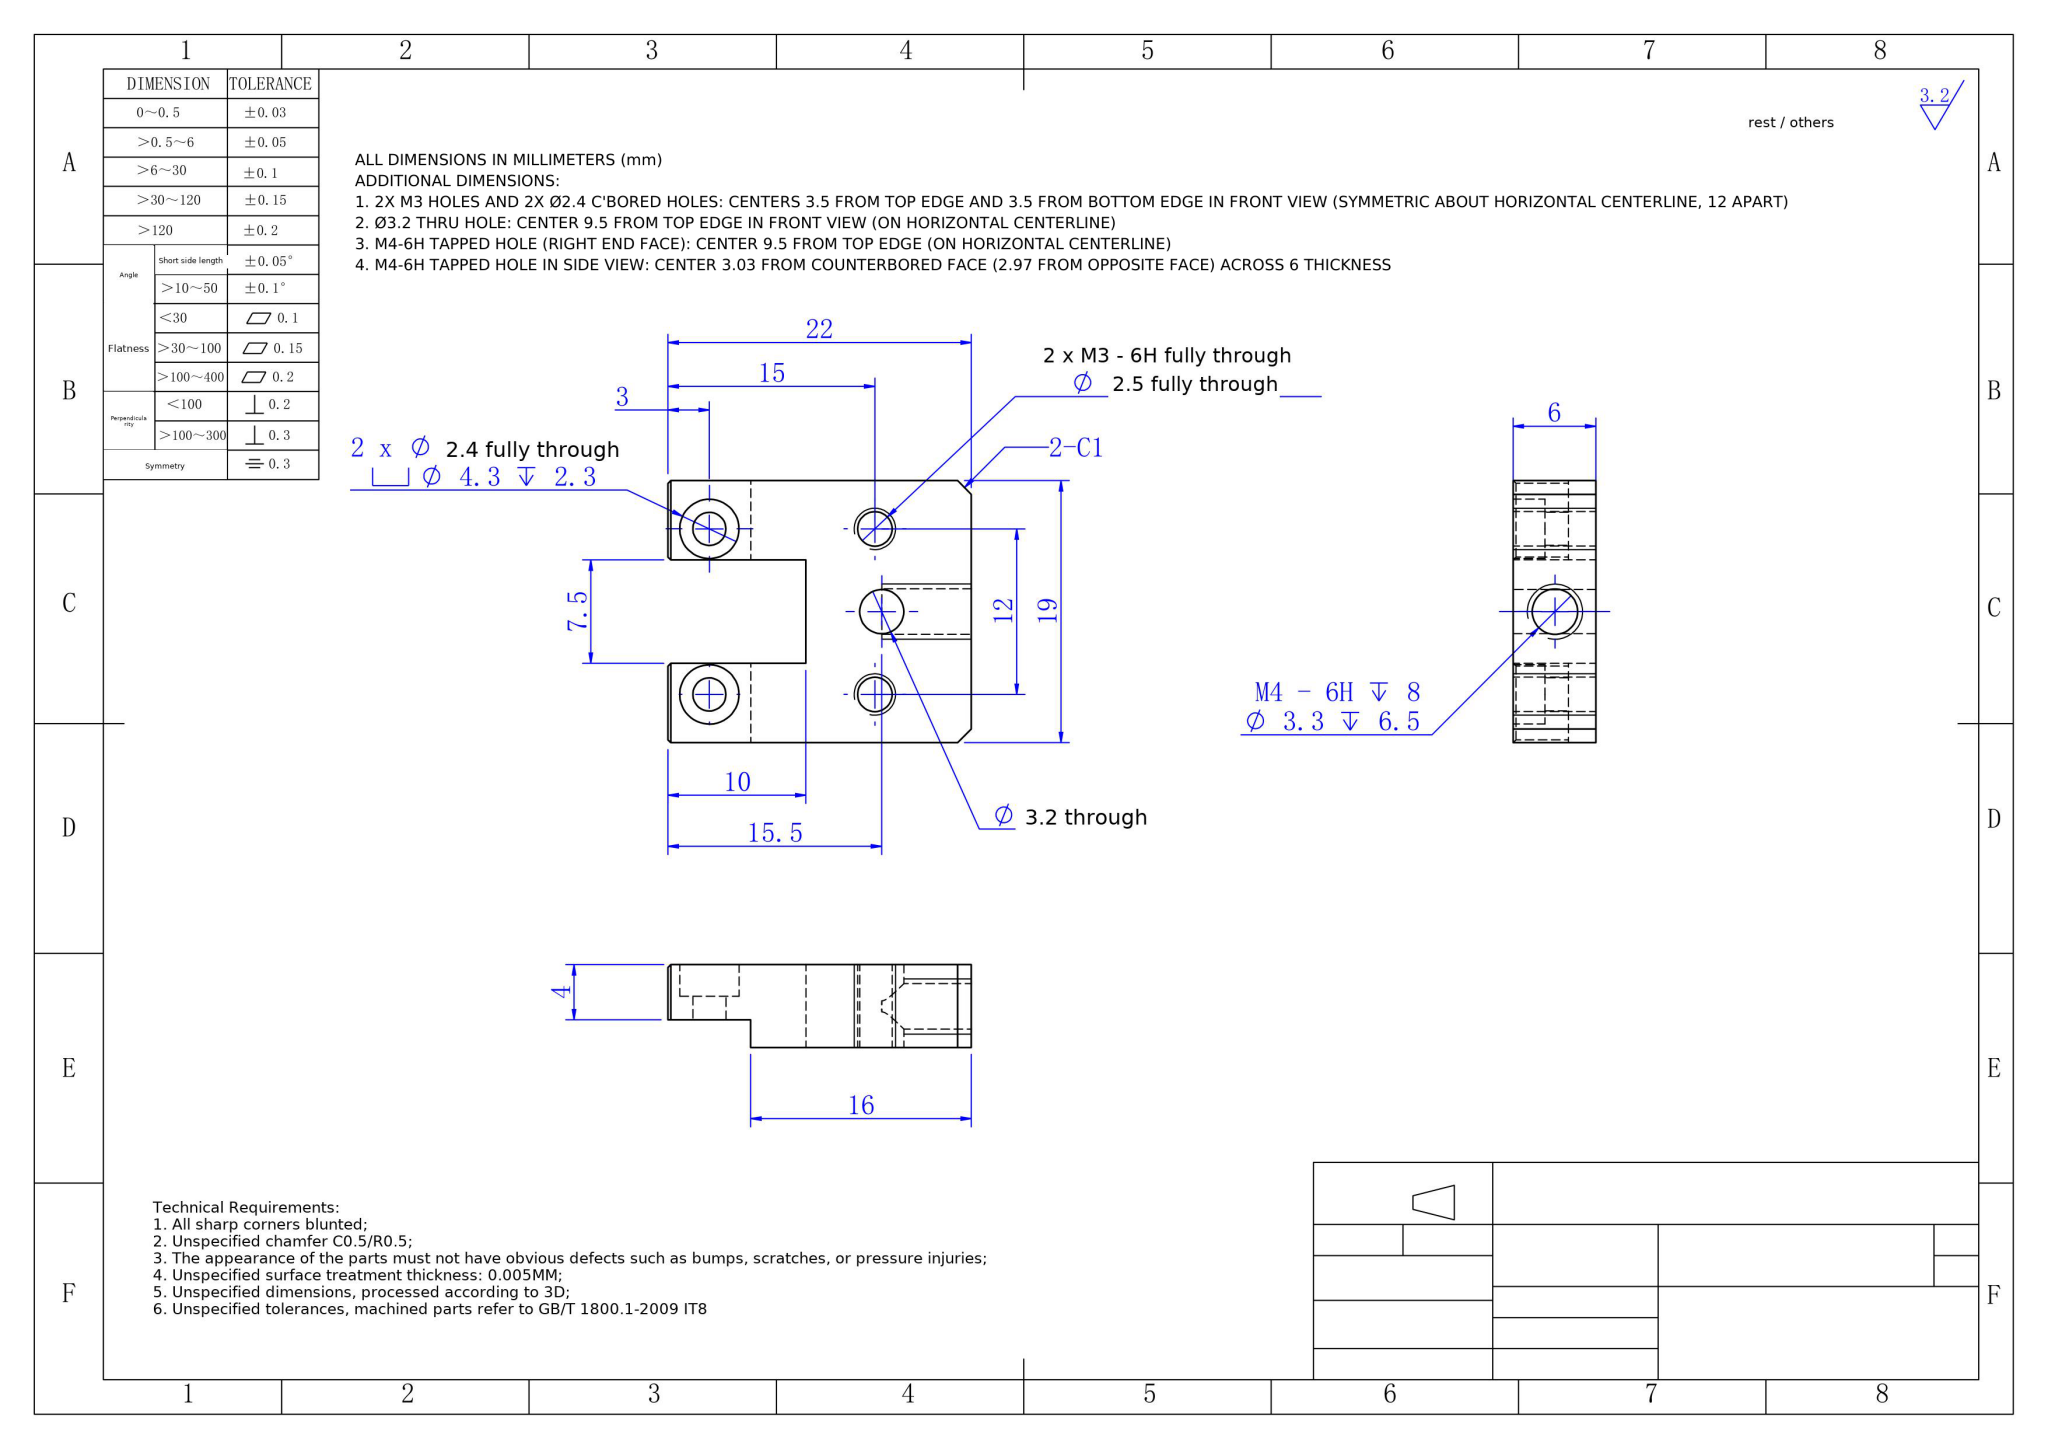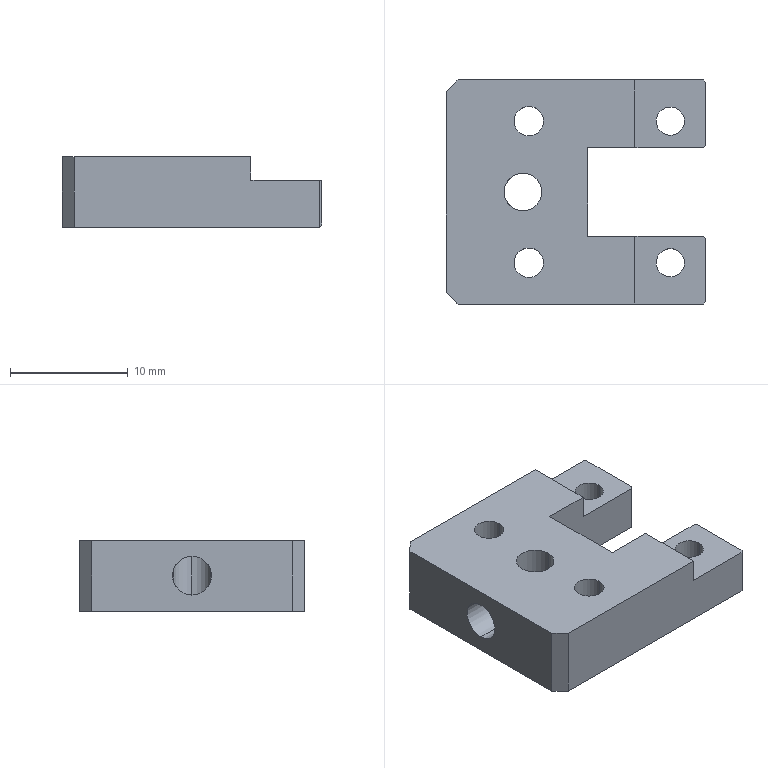Part | NX | mm | 1 solid | 42 faces | box 22 x 19 x 6 mm | volume 1680 mm3 | plane 24 | cylinder 16 | cone 2 | commonest cylinder face diameters 2.5 x4 4.3 x4 2.4 x4 3.3 x2 3.2 x2